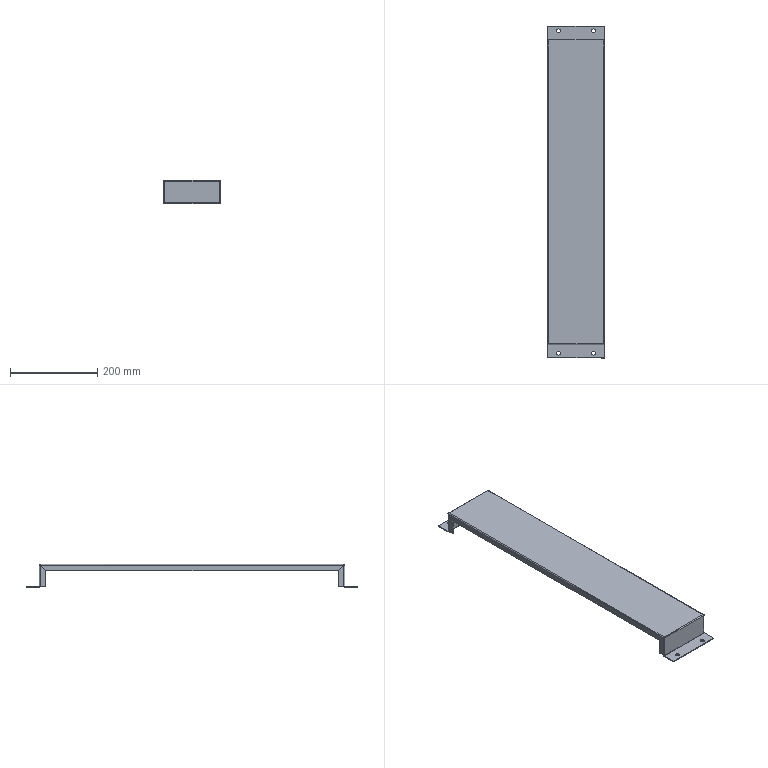Component | SolidWorks | KSHE-016.012-1 | 1 solid | 106 faces | volume 261532 mm3 | plane 70 | cylinder 28 | spline 8 | commonest cylinder face diameters 4.2 x10 0.2 x10 9 x8